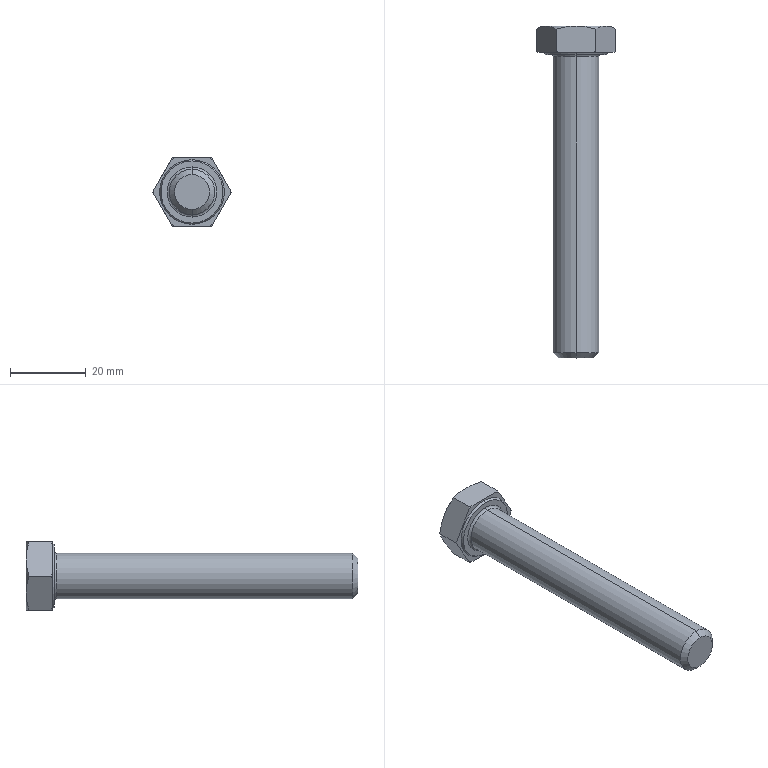Component | SolidWorks | GB_T5780-2016[HexHeadBoltGradeCM12_80]-1 | 1 solid | 30 faces | box 20.78 x 87.5 x 18 mm | volume 11078 mm3 | cone 16 | plane 10 | cylinder 2 | torus 2 | commonest cylinder face diameters 12 x2
build123d program:
from build123d import *

# Parameters (mm, degrees)
BASE_EXTRUDE_DEPTH = 7.5
CHAMFER_2_SIZE     = 1.4


with BuildPart() as part:
    # Sketch1 → Base-Extrude (new body)
    with BuildSketch(Plane(origin=(0, 0, 0), x_dir=(0, 0, -1), z_dir=(1, 0, 0))):
        Polygon((9, 5.196), (9, -5.196), (0, -10.392), (-9, -5.196), (-9, 5.196), (0, 10.392), align=None)
    extrude(amount=BASE_EXTRUDE_DEPTH)

    # Sketch2 → Revolve1 (revolve)
    with BuildSketch(Plane.XY, mode=Mode.PRIVATE) as revolve1_sk:
        Polygon((0, 0), (87.5, 0), (87.5, 4.484), (87.5, 6), (7.5, 6), (0, 6), align=None)
    revolve(revolve1_sk.sketch.rotate(Axis((0, 0, 0), (-1, 0, 0)), 90), axis=Axis((0, 0, 0), (-1, 0, 0)))

    # Sketch3 → Cut-Revolve1 (revolve, cut)
    with BuildSketch(Plane.XY):
        Polygon((0, 9), (3.691, 15.392), (3.691, 20.392), (-10, 20.392), (-10, 9), align=None)
    revolve(axis=Axis((0, 0, 0), (1, 0, 0)), mode=Mode.SUBTRACT)

    # Sketch5 → Cut-Revolve2 (revolve, cut)
    with BuildSketch(Plane.XY):
        Polygon((7.5, 9), (3.809, 15.392), (3.809, 20.392), (13.809, 20.392), (13.809, 9), align=None)
    revolve(axis=Axis((0, 0, 0), (1, 0, 0)), mode=Mode.SUBTRACT)

    # Sketch4 → Cut-Revolve3 (revolve, cut)
    with BuildSketch(Plane.XY, mode=Mode.PRIVATE) as cut_revolve3_sk:
        Polygon((7.5, 8.177), (6.9, 8.524), (6.9, 20.392), (7.5, 20.392), align=None)
    revolve(cut_revolve3_sk.sketch.rotate(Axis((0, 0, 0), (1, 0, 0)), 90), axis=Axis((0, 0, 0), (1, 0, 0)), mode=Mode.SUBTRACT)

    # Chamfer 2
    chamfer_2_edges = [part.edges().sort_by_distance(p)[0] for p in [
        (87.5, 0, 6),
    ]]
    chamfer(chamfer_2_edges, length=CHAMFER_2_SIZE)

    # Sketch9 → Revolve1_2 (revolve)
    with BuildSketch(Plane.XY, mode=Mode.PRIVATE) as revolve1_2_sk:
        with BuildLine():
            Line((7.5, 6.6), (7.5, 6))
            Line((7.5, 6), (8.1, 6))
            ThreePointArc((8.1, 6), (7.676, 6.176), (7.5, 6.6))
        make_face()
    revolve(revolve1_2_sk.sketch.rotate(Axis((0, 0, 0), (1, 0, 0)), 90), axis=Axis((0, 0, 0), (1, 0, 0)))


solid = part.part

# Placed as in the assembly
solid = solid.moved(Location((-380, 37.5, 90), (0, 0, -90)))
STEP:
#1=COLOUR_RGB('',0.7922,0.8196,0.9333);
#2=FILL_AREA_STYLE_COLOUR('',#1);
#3=FILL_AREA_STYLE('',(#2));
#4=SURFACE_STYLE_FILL_AREA(#3);
#5=SURFACE_SIDE_STYLE('',(#4));
#6=SURFACE_STYLE_USAGE(.BOTH.,#5);
#7=PRESENTATION_STYLE_ASSIGNMENT((#6));
#8=CARTESIAN_POINT('',(-14.961,1.157,3.78));
#9=VERTEX_POINT('',#8);
#10=CARTESIAN_POINT('',(-14.961,1.157,3.307));
#11=VERTEX_POINT('',#10);
#12=CARTESIAN_POINT('',(-14.961,1.157,3.543));
#13=DIRECTION('',(-0.,1.,0.));
#14=DIRECTION('',(0.,0.,1.));
#15=AXIS2_PLACEMENT_3D('',#12,#13,#14);
#16=CIRCLE('',#15,0.2362);
#17=EDGE_CURVE('',#9,#11,#16,.T.);
#18=ORIENTED_EDGE('',*,*,#17,.F.);
#19=CARTESIAN_POINT('',(-14.961,-1.913,3.78));
#20=VERTEX_POINT('',#19);
#21=CARTESIAN_POINT('',(-14.961,1.476,3.78));
#22=DIRECTION('',(0.,-1.,0.));
#23=VECTOR('',#22,39.37);
#24=LINE('',#21,#23);
#25=EDGE_CURVE('',#9,#20,#24,.T.);
#26=ORIENTED_EDGE('',*,*,#25,.T.);
#27=CARTESIAN_POINT('',(-14.961,-1.913,3.307));
#28=VERTEX_POINT('',#27);
#29=CARTESIAN_POINT('',(-14.961,-1.913,3.543));
#30=DIRECTION('',(-0.,1.,0.));
#31=DIRECTION('',(-0.,0.,-1.));
#32=AXIS2_PLACEMENT_3D('',#29,#30,#31);
#33=CIRCLE('',#32,0.2362);
#34=EDGE_CURVE('',#20,#28,#33,.T.);
#35=ORIENTED_EDGE('',*,*,#34,.T.);
#36=CARTESIAN_POINT('',(-14.961,1.476,3.307));
#37=DIRECTION('',(0.,-1.,0.));
#38=VECTOR('',#37,39.37);
#39=LINE('',#36,#38);
#40=EDGE_CURVE('',#11,#28,#39,.T.);
#41=ORIENTED_EDGE('',*,*,#40,.F.);
#42=EDGE_LOOP('',(#18,#26,#35,#41));
#43=FACE_OUTER_BOUND('',#42,.T.);
#44=CARTESIAN_POINT('',(-14.961,1.476,3.543));
#45=DIRECTION('',(0.,-1.,0.));
#46=DIRECTION('',(0.,0.,-1.));
#47=AXIS2_PLACEMENT_3D('',#44,#45,#46);
#48=CYLINDRICAL_SURFACE('',#47,0.2362);
#49=ADVANCED_FACE('',(#43),#48,.T.);
#50=CARTESIAN_POINT('',(-14.961,-1.969,3.362));
#51=VERTEX_POINT('',#50);
#52=CARTESIAN_POINT('',(-14.961,-1.969,3.724));
#53=VERTEX_POINT('',#52);
#54=CARTESIAN_POINT('',(-14.961,-1.969,3.543));
#55=DIRECTION('',(0.,-1.,0.));
#56=DIRECTION('',(0.,0.,-1.));
#57=AXIS2_PLACEMENT_3D('',#54,#55,#56);
#58=CIRCLE('',#57,0.1811);
#59=EDGE_CURVE('',#51,#53,#58,.T.);
#60=ORIENTED_EDGE('',*,*,#59,.F.);
#61=CARTESIAN_POINT('',(-14.961,-1.969,3.362));
#62=DIRECTION('',(-0.,0.7071,-0.7071));
#63=VECTOR('',#62,39.37);
#64=LINE('',#61,#63);
#65=EDGE_CURVE('',#51,#28,#64,.T.);
#66=ORIENTED_EDGE('',*,*,#65,.T.);
#67=ORIENTED_EDGE('',*,*,#34,.F.);
#68=CARTESIAN_POINT('',(-14.961,-1.969,3.724));
#69=DIRECTION('',(-0.,0.7071,0.7071));
#70=VECTOR('',#69,39.37);
#71=LINE('',#68,#70);
#72=EDGE_CURVE('',#53,#20,#71,.T.);
#73=ORIENTED_EDGE('',*,*,#72,.F.);
#74=EDGE_LOOP('',(#60,#66,#67,#73));
#75=FACE_OUTER_BOUND('',#74,.T.);
#76=CARTESIAN_POINT('',(-14.961,-1.969,3.543));
#77=DIRECTION('',(-0.,1.,0.));
#78=DIRECTION('',(0.,0.,1.));
#79=AXIS2_PLACEMENT_3D('',#76,#77,#78);
#80=CONICAL_SURFACE('',#79,0.1811,0.7854);
#81=ADVANCED_FACE('',(#75),#80,.T.);
#82=CARTESIAN_POINT('',(-14.961,1.181,3.283));
#83=VERTEX_POINT('',#82);
#84=CARTESIAN_POINT('',(-14.961,1.181,3.803));
#85=VERTEX_POINT('',#84);
#86=CARTESIAN_POINT('',(-14.961,1.181,3.543));
#87=DIRECTION('',(-0.,1.,0.));
#88=DIRECTION('',(0.,0.,1.));
#89=AXIS2_PLACEMENT_3D('',#86,#87,#88);
#90=CIRCLE('',#89,0.2598);
#91=EDGE_CURVE('',#83,#85,#90,.T.);
#92=ORIENTED_EDGE('',*,*,#91,.F.);
#93=CARTESIAN_POINT('',(-14.961,1.157,3.283));
#94=DIRECTION('',(1.,0.,0.));
#95=DIRECTION('',(0.,1.,0.));
#96=AXIS2_PLACEMENT_3D('',#93,#94,#95);
#97=CIRCLE('',#96,0.02362);
#98=EDGE_CURVE('',#83,#11,#97,.T.);
#99=ORIENTED_EDGE('',*,*,#98,.T.);
#100=CARTESIAN_POINT('',(-14.961,1.157,3.543));
#101=DIRECTION('',(-0.,1.,0.));
#102=DIRECTION('',(0.,0.,1.));
#103=AXIS2_PLACEMENT_3D('',#100,#101,#102);
#104=CIRCLE('',#103,0.2362);
#105=EDGE_CURVE('',#11,#9,#104,.T.);
#106=ORIENTED_EDGE('',*,*,#105,.T.);
#107=CARTESIAN_POINT('',(-14.961,1.157,3.803));
#108=DIRECTION('',(-1.,-0.,0.));
#109=DIRECTION('',(0.,-1.,0.));
#110=AXIS2_PLACEMENT_3D('',#107,#108,#109);
#111=CIRCLE('',#110,0.02362);
#112=EDGE_CURVE('',#85,#9,#111,.T.);
#113=ORIENTED_EDGE('',*,*,#112,.F.);
#114=EDGE_LOOP('',(#92,#99,#106,#113));
#115=FACE_OUTER_BOUND('',#114,.T.);
#116=CARTESIAN_POINT('',(-14.961,1.157,3.543));
#117=DIRECTION('',(-0.,1.,0.));
#118=DIRECTION('',(0.,0.,1.));
#119=AXIS2_PLACEMENT_3D('',#116,#117,#118);
#120=TOROIDAL_SURFACE('',#119,0.2598,0.02362);
#121=ADVANCED_FACE('',(#115),#120,.F.);
#122=CARTESIAN_POINT('',(-14.961,1.181,3.865));
#123=VERTEX_POINT('',#122);
#124=CARTESIAN_POINT('',(-14.961,1.181,3.221));
#125=VERTEX_POINT('',#124);
#126=CARTESIAN_POINT('',(-14.961,1.181,3.543));
#127=DIRECTION('',(-0.,1.,0.));
#128=DIRECTION('',(0.,0.,1.));
#129=AXIS2_PLACEMENT_3D('',#126,#127,#128);
#130=CIRCLE('',#129,0.3219);
#131=EDGE_CURVE('',#123,#125,#130,.T.);
#132=ORIENTED_EDGE('',*,*,#131,.T.);
#133=CARTESIAN_POINT('',(-14.961,1.205,3.208));
#134=VERTEX_POINT('',#133);
#135=CARTESIAN_POINT('',(-14.961,1.205,3.208));
#136=DIRECTION('',(-0.,0.866,-0.5));
#137=VECTOR('',#136,39.37);
#138=LINE('',#135,#137);
#139=EDGE_CURVE('',#125,#134,#138,.T.);
#140=ORIENTED_EDGE('',*,*,#139,.T.);
#141=CARTESIAN_POINT('',(-14.961,1.205,3.879));
#142=VERTEX_POINT('',#141);
#143=CARTESIAN_POINT('',(-14.961,1.205,3.543));
#144=DIRECTION('',(-0.,1.,0.));
#145=DIRECTION('',(0.,0.,1.));
#146=AXIS2_PLACEMENT_3D('',#143,#144,#145);
#147=CIRCLE('',#146,0.3356);
#148=EDGE_CURVE('',#142,#134,#147,.T.);
#149=ORIENTED_EDGE('',*,*,#148,.F.);
#150=CARTESIAN_POINT('',(-14.961,1.205,3.879));
#151=DIRECTION('',(-0.,0.866,0.5));
#152=VECTOR('',#151,39.37);
#153=LINE('',#150,#152);
#154=EDGE_CURVE('',#123,#142,#153,.T.);
#155=ORIENTED_EDGE('',*,*,#154,.F.);
#156=EDGE_LOOP('',(#132,#140,#149,#155));
#157=FACE_OUTER_BOUND('',#156,.T.);
#158=CARTESIAN_POINT('',(-14.961,1.205,3.543));
#159=DIRECTION('',(-0.,1.,0.));
#160=DIRECTION('',(0.,0.,1.));
#161=AXIS2_PLACEMENT_3D('',#158,#159,#160);
#162=CONICAL_SURFACE('',#161,0.3356,0.5236);
#163=ADVANCED_FACE('',(#157),#162,.T.);
#164=ORIENTED_EDGE('',*,*,#131,.F.);
#165=CARTESIAN_POINT('',(-14.961,1.181,3.543));
#166=DIRECTION('',(-0.,1.,0.));
#167=DIRECTION('',(0.,0.,1.));
#168=AXIS2_PLACEMENT_3D('',#165,#166,#167);
#169=CIRCLE('',#168,0.3219);
#170=EDGE_CURVE('',#125,#123,#169,.T.);
#171=ORIENTED_EDGE('',*,*,#170,.F.);
#172=EDGE_LOOP('',(#164,#171));
#173=FACE_OUTER_BOUND('',#172,.T.);
#174=CARTESIAN_POINT('',(-14.961,1.181,3.543));
#175=DIRECTION('',(-0.,1.,0.));
#176=DIRECTION('',(0.,0.,1.));
#177=AXIS2_PLACEMENT_3D('',#174,#175,#176);
#178=CIRCLE('',#177,0.2598);
#179=EDGE_CURVE('',#85,#83,#178,.T.);
#180=ORIENTED_EDGE('',*,*,#179,.T.);
#181=ORIENTED_EDGE('',*,*,#91,.T.);
#182=EDGE_LOOP('',(#180,#181));
#183=FACE_BOUND('',#182,.T.);
#184=CARTESIAN_POINT('',(-14.551,1.181,3.543));
#185=DIRECTION('',(0.,-1.,0.));
#186=DIRECTION('',(0.,0.,-1.));
#187=AXIS2_PLACEMENT_3D('',#184,#185,#186);
#188=PLANE('',#187);
#189=ADVANCED_FACE('',(#173,#183),#188,.T.);
#190=CARTESIAN_POINT('',(-14.741,1.205,3.214));
#191=VERTEX_POINT('',#190);
#192=CARTESIAN_POINT('',(-14.566,1.205,3.518));
#193=VERTEX_POINT('',#192);
#194=CARTESIAN_POINT('',(-14.756,1.205,3.189));
#195=DIRECTION('',(0.5,0.,0.866));
#196=VECTOR('',#195,39.37);
#197=LINE('',#194,#196);
#198=EDGE_CURVE('',#191,#193,#197,.T.);
#199=ORIENTED_EDGE('',*,*,#198,.F.);
#200=CARTESIAN_POINT('',(-14.756,1.213,3.189));
#201=VERTEX_POINT('',#200);
#202=CARTESIAN_POINT('',(-14.756,1.213,3.189));
#203=CARTESIAN_POINT('',(-14.751,1.21,3.197));
#204=CARTESIAN_POINT('',(-14.746,1.207,3.206));
#205=CARTESIAN_POINT('',(-14.741,1.205,3.214));
#206=B_SPLINE_CURVE_WITH_KNOTS('',3,(#202,#203,#204,#205),.UNSPECIFIED.,.F.,.F.,(4,4),(0.00000024,0.0007696),.UNSPECIFIED.);
#207=EDGE_CURVE('',#201,#191,#206,.T.);
#208=ORIENTED_EDGE('',*,*,#207,.F.);
#209=CARTESIAN_POINT('',(-14.756,1.445,3.189));
#210=VERTEX_POINT('',#209);
#211=CARTESIAN_POINT('',(-14.756,1.181,3.189));
#212=DIRECTION('',(-0.,1.,0.));
#213=VECTOR('',#212,39.37);
#214=LINE('',#211,#213);
#215=EDGE_CURVE('',#201,#210,#214,.T.);
#216=ORIENTED_EDGE('',*,*,#215,.T.);
#217=CARTESIAN_POINT('',(-14.654,1.476,3.366));
#218=VERTEX_POINT('',#217);
#219=CARTESIAN_POINT('',(-14.654,1.476,3.366));
#220=CARTESIAN_POINT('',(-14.662,1.476,3.351));
#221=CARTESIAN_POINT('',(-14.671,1.476,3.336));
#222=CARTESIAN_POINT('',(-14.688,1.473,3.306));
#223=CARTESIAN_POINT('',(-14.697,1.471,3.291));
#224=CARTESIAN_POINT('',(-14.723,1.462,3.247));
#225=CARTESIAN_POINT('',(-14.739,1.454,3.218));
#226=CARTESIAN_POINT('',(-14.756,1.445,3.189));
#227=B_SPLINE_CURVE_WITH_KNOTS('',3,(#219,#220,#221,#222,#223,#224,#225,#226),.UNSPECIFIED.,.F.,.F.,(4,2,2,4),(0.005258,0.006567,0.007877,0.0105),.UNSPECIFIED.);
#228=EDGE_CURVE('',#218,#210,#227,.T.);
#229=ORIENTED_EDGE('',*,*,#228,.F.);
#230=CARTESIAN_POINT('',(-14.551,1.445,3.543));
#231=VERTEX_POINT('',#230);
#232=CARTESIAN_POINT('',(-14.551,1.445,3.543));
#233=CARTESIAN_POINT('',(-14.568,1.454,3.514));
#234=CARTESIAN_POINT('',(-14.585,1.462,3.485));
#235=CARTESIAN_POINT('',(-14.619,1.473,3.426));
#236=CARTESIAN_POINT('',(-14.636,1.476,3.396));
#237=CARTESIAN_POINT('',(-14.654,1.476,3.366));
#238=B_SPLINE_CURVE_WITH_KNOTS('',3,(#232,#233,#234,#235,#236,#237),.UNSPECIFIED.,.F.,.F.,(4,2,4),(0.00000024,0.002629,0.005258),.UNSPECIFIED.);
#239=EDGE_CURVE('',#231,#218,#238,.T.);
#240=ORIENTED_EDGE('',*,*,#239,.F.);
#241=CARTESIAN_POINT('',(-14.551,1.213,3.543));
#242=VERTEX_POINT('',#241);
#243=CARTESIAN_POINT('',(-14.551,1.181,3.543));
#244=DIRECTION('',(-0.,1.,0.));
#245=VECTOR('',#244,39.37);
#246=LINE('',#243,#245);
#247=EDGE_CURVE('',#242,#231,#246,.T.);
#248=ORIENTED_EDGE('',*,*,#247,.F.);
#249=CARTESIAN_POINT('',(-14.566,1.205,3.518));
#250=CARTESIAN_POINT('',(-14.561,1.207,3.526));
#251=CARTESIAN_POINT('',(-14.556,1.21,3.535));
#252=CARTESIAN_POINT('',(-14.551,1.213,3.543));
#253=B_SPLINE_CURVE_WITH_KNOTS('',3,(#249,#250,#251,#252),.UNSPECIFIED.,.F.,.F.,(4,4),(0.009728,0.0105),.UNSPECIFIED.);
#254=EDGE_CURVE('',#193,#242,#253,.T.);
#255=ORIENTED_EDGE('',*,*,#254,.F.);
#256=EDGE_LOOP('',(#199,#208,#216,#229,#240,#248,#255));
#257=FACE_OUTER_BOUND('',#256,.T.);
#258=CARTESIAN_POINT('',(-14.756,1.181,3.189));
#259=DIRECTION('',(-0.866,-0.,0.5));
#260=DIRECTION('',(-0.5,-0.,-0.866));
#261=AXIS2_PLACEMENT_3D('',#258,#259,#260);
#262=PLANE('',#261);
#263=ADVANCED_FACE('',(#257),#262,.F.);
#264=CARTESIAN_POINT('',(-14.566,1.205,3.569));
#265=VERTEX_POINT('',#264);
#266=CARTESIAN_POINT('',(-14.741,1.205,3.872));
#267=VERTEX_POINT('',#266);
#268=CARTESIAN_POINT('',(-14.551,1.205,3.543));
#269=DIRECTION('',(-0.5,-0.,0.866));
#270=VECTOR('',#269,39.37);
#271=LINE('',#268,#270);
#272=EDGE_CURVE('',#265,#267,#271,.T.);
#273=ORIENTED_EDGE('',*,*,#272,.F.);
#274=CARTESIAN_POINT('',(-14.551,1.213,3.543));
#275=CARTESIAN_POINT('',(-14.556,1.21,3.552));
#276=CARTESIAN_POINT('',(-14.561,1.207,3.56));
#277=CARTESIAN_POINT('',(-14.566,1.205,3.569));
#278=B_SPLINE_CURVE_WITH_KNOTS('',3,(#274,#275,#276,#277),.UNSPECIFIED.,.F.,.F.,(4,4),(0.00000024,0.0007696),.UNSPECIFIED.);
#279=EDGE_CURVE('',#242,#265,#278,.T.);
#280=ORIENTED_EDGE('',*,*,#279,.F.);
#281=ORIENTED_EDGE('',*,*,#247,.T.);
#282=CARTESIAN_POINT('',(-14.654,1.476,3.72));
#283=VERTEX_POINT('',#282);
#284=CARTESIAN_POINT('',(-14.654,1.476,3.72));
#285=CARTESIAN_POINT('',(-14.645,1.476,3.705));
#286=CARTESIAN_POINT('',(-14.636,1.476,3.69));
#287=CARTESIAN_POINT('',(-14.619,1.473,3.66));
#288=CARTESIAN_POINT('',(-14.611,1.471,3.646));
#289=CARTESIAN_POINT('',(-14.585,1.462,3.601));
#290=CARTESIAN_POINT('',(-14.568,1.454,3.572));
#291=CARTESIAN_POINT('',(-14.551,1.445,3.543));
#292=B_SPLINE_CURVE_WITH_KNOTS('',3,(#284,#285,#286,#287,#288,#289,#290,#291),.UNSPECIFIED.,.F.,.F.,(4,2,2,4),(0.005258,0.006567,0.007877,0.0105),.UNSPECIFIED.);
#293=EDGE_CURVE('',#283,#231,#292,.T.);
#294=ORIENTED_EDGE('',*,*,#293,.F.);
#295=CARTESIAN_POINT('',(-14.756,1.445,3.898));
#296=VERTEX_POINT('',#295);
#297=CARTESIAN_POINT('',(-14.756,1.445,3.898));
#298=CARTESIAN_POINT('',(-14.739,1.454,3.869));
#299=CARTESIAN_POINT('',(-14.722,1.462,3.839));
#300=CARTESIAN_POINT('',(-14.688,1.473,3.78));
#301=CARTESIAN_POINT('',(-14.671,1.476,3.751));
#302=CARTESIAN_POINT('',(-14.654,1.476,3.72));
#303=B_SPLINE_CURVE_WITH_KNOTS('',3,(#297,#298,#299,#300,#301,#302),.UNSPECIFIED.,.F.,.F.,(4,2,4),(0.00000024,0.002629,0.005258),.UNSPECIFIED.);
#304=EDGE_CURVE('',#296,#283,#303,.T.);
#305=ORIENTED_EDGE('',*,*,#304,.F.);
#306=CARTESIAN_POINT('',(-14.756,1.213,3.898));
#307=VERTEX_POINT('',#306);
#308=CARTESIAN_POINT('',(-14.756,1.181,3.898));
#309=DIRECTION('',(-0.,1.,0.));
#310=VECTOR('',#309,39.37);
#311=LINE('',#308,#310);
#312=EDGE_CURVE('',#307,#296,#311,.T.);
#313=ORIENTED_EDGE('',*,*,#312,.F.);
#314=CARTESIAN_POINT('',(-14.741,1.205,3.872));
#315=CARTESIAN_POINT('',(-14.746,1.207,3.881));
#316=CARTESIAN_POINT('',(-14.751,1.21,3.889));
#317=CARTESIAN_POINT('',(-14.756,1.213,3.898));
#318=B_SPLINE_CURVE_WITH_KNOTS('',3,(#314,#315,#316,#317),.UNSPECIFIED.,.F.,.F.,(4,4),(0.009728,0.0105),.UNSPECIFIED.);
#319=EDGE_CURVE('',#267,#307,#318,.T.);
#320=ORIENTED_EDGE('',*,*,#319,.F.);
#321=EDGE_LOOP('',(#273,#280,#281,#294,#305,#313,#320));
#322=FACE_OUTER_BOUND('',#321,.T.);
#323=CARTESIAN_POINT('',(-14.551,1.181,3.543));
#324=DIRECTION('',(-0.866,-0.,-0.5));
#325=DIRECTION('',(0.5,0.,-0.866));
#326=AXIS2_PLACEMENT_3D('',#323,#324,#325);
#327=PLANE('',#326);
#328=ADVANCED_FACE('',(#322),#327,.F.);
#329=CARTESIAN_POINT('',(-14.786,1.205,3.898));
#330=VERTEX_POINT('',#329);
#331=CARTESIAN_POINT('',(-15.136,1.205,3.898));
#332=VERTEX_POINT('',#331);
#333=CARTESIAN_POINT('',(-14.756,1.205,3.898));
#334=DIRECTION('',(-1.,-0.,-0.));
#335=VECTOR('',#334,39.37);
#336=LINE('',#333,#335);
#337=EDGE_CURVE('',#330,#332,#336,.T.);
#338=ORIENTED_EDGE('',*,*,#337,.F.);
#339=CARTESIAN_POINT('',(-14.756,1.213,3.898));
#340=CARTESIAN_POINT('',(-14.766,1.21,3.898));
#341=CARTESIAN_POINT('',(-14.776,1.207,3.898));
#342=CARTESIAN_POINT('',(-14.786,1.205,3.898));
#343=B_SPLINE_CURVE_WITH_KNOTS('',3,(#339,#340,#341,#342),.UNSPECIFIED.,.F.,.F.,(4,4),(0.02519,0.02597),.UNSPECIFIED.);
#344=EDGE_CURVE('',#307,#330,#343,.T.);
#345=ORIENTED_EDGE('',*,*,#344,.F.);
#346=ORIENTED_EDGE('',*,*,#312,.T.);
#347=CARTESIAN_POINT('',(-14.961,1.476,3.898));
#348=VERTEX_POINT('',#347);
#349=CARTESIAN_POINT('',(-14.961,1.476,3.898));
#350=CARTESIAN_POINT('',(-14.943,1.476,3.898));
#351=CARTESIAN_POINT('',(-14.926,1.476,3.898));
#352=CARTESIAN_POINT('',(-14.891,1.473,3.898));
#353=CARTESIAN_POINT('',(-14.874,1.471,3.898));
#354=CARTESIAN_POINT('',(-14.823,1.462,3.898));
#355=CARTESIAN_POINT('',(-14.789,1.454,3.898));
#356=CARTESIAN_POINT('',(-14.756,1.445,3.898));
#357=B_SPLINE_CURVE_WITH_KNOTS('',3,(#349,#350,#351,#352,#353,#354,#355,#356),.UNSPECIFIED.,.F.,.F.,(4,2,2,4),(0.01498,0.0163,0.01761,0.02025),.UNSPECIFIED.);
#358=EDGE_CURVE('',#348,#296,#357,.T.);
#359=ORIENTED_EDGE('',*,*,#358,.F.);
#360=CARTESIAN_POINT('',(-15.165,1.445,3.898));
#361=VERTEX_POINT('',#360);
#362=CARTESIAN_POINT('',(-15.165,1.445,3.898));
#363=CARTESIAN_POINT('',(-15.132,1.454,3.898));
#364=CARTESIAN_POINT('',(-15.098,1.462,3.898));
#365=CARTESIAN_POINT('',(-15.03,1.473,3.898));
#366=CARTESIAN_POINT('',(-14.995,1.476,3.898));
#367=CARTESIAN_POINT('',(-14.961,1.476,3.898));
#368=B_SPLINE_CURVE_WITH_KNOTS('',3,(#362,#363,#364,#365,#366,#367),.UNSPECIFIED.,.F.,.F.,(4,2,4),(0.00972,0.01235,0.01498),.UNSPECIFIED.);
#369=EDGE_CURVE('',#361,#348,#368,.T.);
#370=ORIENTED_EDGE('',*,*,#369,.F.);
#371=CARTESIAN_POINT('',(-15.165,1.213,3.898));
#372=VERTEX_POINT('',#371);
#373=CARTESIAN_POINT('',(-15.165,1.181,3.898));
#374=DIRECTION('',(-0.,1.,0.));
#375=VECTOR('',#374,39.37);
#376=LINE('',#373,#375);
#377=EDGE_CURVE('',#372,#361,#376,.T.);
#378=ORIENTED_EDGE('',*,*,#377,.F.);
#379=CARTESIAN_POINT('',(-15.136,1.205,3.898));
#380=CARTESIAN_POINT('',(-15.146,1.207,3.898));
#381=CARTESIAN_POINT('',(-15.155,1.21,3.898));
#382=CARTESIAN_POINT('',(-15.165,1.213,3.898));
#383=B_SPLINE_CURVE_WITH_KNOTS('',3,(#379,#380,#381,#382),.UNSPECIFIED.,.F.,.F.,(4,4),(0.03494,0.03571),.UNSPECIFIED.);
#384=EDGE_CURVE('',#332,#372,#383,.T.);
#385=ORIENTED_EDGE('',*,*,#384,.F.);
#386=EDGE_LOOP('',(#338,#345,#346,#359,#370,#378,#385));
#387=FACE_OUTER_BOUND('',#386,.T.);
#388=CARTESIAN_POINT('',(-14.756,1.181,3.898));
#389=DIRECTION('',(0.,0.,-1.));
#390=DIRECTION('',(1.,0.,0.));
#391=AXIS2_PLACEMENT_3D('',#388,#389,#390);
#392=PLANE('',#391);
#393=ADVANCED_FACE('',(#387),#392,.F.);
#394=CARTESIAN_POINT('',(-15.18,1.205,3.872));
#395=VERTEX_POINT('',#394);
#396=CARTESIAN_POINT('',(-15.355,1.205,3.569));
#397=VERTEX_POINT('',#396);
#398=CARTESIAN_POINT('',(-15.37,1.205,3.543));
#399=DIRECTION('',(-0.5,-0.,-0.866));
#400=VECTOR('',#399,39.37);
#401=LINE('',#398,#400);
#402=EDGE_CURVE('',#395,#397,#401,.T.);
#403=ORIENTED_EDGE('',*,*,#402,.F.);
#404=CARTESIAN_POINT('',(-15.165,1.213,3.898));
#405=CARTESIAN_POINT('',(-15.17,1.21,3.889));
#406=CARTESIAN_POINT('',(-15.175,1.207,3.881));
#407=CARTESIAN_POINT('',(-15.18,1.205,3.872));
#408=B_SPLINE_CURVE_WITH_KNOTS('',3,(#404,#405,#406,#407),.UNSPECIFIED.,.F.,.F.,(4,4),(0.00000024,0.0007696),.UNSPECIFIED.);
#409=EDGE_CURVE('',#372,#395,#408,.T.);
#410=ORIENTED_EDGE('',*,*,#409,.F.);
#411=ORIENTED_EDGE('',*,*,#377,.T.);
#412=CARTESIAN_POINT('',(-15.267,1.476,3.72));
#413=VERTEX_POINT('',#412);
#414=CARTESIAN_POINT('',(-15.267,1.476,3.72));
#415=CARTESIAN_POINT('',(-15.259,1.476,3.736));
#416=CARTESIAN_POINT('',(-15.25,1.476,3.751));
#417=CARTESIAN_POINT('',(-15.233,1.473,3.78));
#418=CARTESIAN_POINT('',(-15.224,1.471,3.795));
#419=CARTESIAN_POINT('',(-15.199,1.462,3.84));
#420=CARTESIAN_POINT('',(-15.182,1.454,3.869));
#421=CARTESIAN_POINT('',(-15.165,1.445,3.898));
#422=B_SPLINE_CURVE_WITH_KNOTS('',3,(#414,#415,#416,#417,#418,#419,#420,#421),.UNSPECIFIED.,.F.,.F.,(4,2,2,4),(0.005258,0.006567,0.007877,0.0105),.UNSPECIFIED.);
#423=EDGE_CURVE('',#413,#361,#422,.T.);
#424=ORIENTED_EDGE('',*,*,#423,.F.);
#425=CARTESIAN_POINT('',(-15.37,1.445,3.543));
#426=VERTEX_POINT('',#425);
#427=CARTESIAN_POINT('',(-15.37,1.445,3.543));
#428=CARTESIAN_POINT('',(-15.353,1.454,3.572));
#429=CARTESIAN_POINT('',(-15.336,1.462,3.601));
#430=CARTESIAN_POINT('',(-15.302,1.473,3.66));
#431=CARTESIAN_POINT('',(-15.285,1.476,3.69));
#432=CARTESIAN_POINT('',(-15.267,1.476,3.72));
#433=B_SPLINE_CURVE_WITH_KNOTS('',3,(#427,#428,#429,#430,#431,#432),.UNSPECIFIED.,.F.,.F.,(4,2,4),(0.00000024,0.002629,0.005258),.UNSPECIFIED.);
#434=EDGE_CURVE('',#426,#413,#433,.T.);
#435=ORIENTED_EDGE('',*,*,#434,.F.);
#436=CARTESIAN_POINT('',(-15.37,1.213,3.543));
#437=VERTEX_POINT('',#436);
#438=CARTESIAN_POINT('',(-15.37,1.181,3.543));
#439=DIRECTION('',(-0.,1.,0.));
#440=VECTOR('',#439,39.37);
#441=LINE('',#438,#440);
#442=EDGE_CURVE('',#437,#426,#441,.T.);
#443=ORIENTED_EDGE('',*,*,#442,.F.);
#444=CARTESIAN_POINT('',(-15.355,1.205,3.569));
#445=CARTESIAN_POINT('',(-15.36,1.207,3.56));
#446=CARTESIAN_POINT('',(-15.365,1.21,3.552));
#447=CARTESIAN_POINT('',(-15.37,1.213,3.543));
#448=B_SPLINE_CURVE_WITH_KNOTS('',3,(#444,#445,#446,#447),.UNSPECIFIED.,.F.,.F.,(4,4),(0.009728,0.0105),.UNSPECIFIED.);
#449=EDGE_CURVE('',#397,#437,#448,.T.);
#450=ORIENTED_EDGE('',*,*,#449,.F.);
#451=EDGE_LOOP('',(#403,#410,#411,#424,#435,#443,#450));
#452=FACE_OUTER_BOUND('',#451,.T.);
#453=CARTESIAN_POINT('',(-15.37,1.181,3.543));
#454=DIRECTION('',(0.866,0.,-0.5));
#455=DIRECTION('',(0.5,0.,0.866));
#456=AXIS2_PLACEMENT_3D('',#453,#454,#455);
#457=PLANE('',#456);
#458=ADVANCED_FACE('',(#452),#457,.F.);
#459=CARTESIAN_POINT('',(-15.355,1.205,3.518));
#460=VERTEX_POINT('',#459);
#461=CARTESIAN_POINT('',(-15.18,1.205,3.214));
#462=VERTEX_POINT('',#461);
#463=CARTESIAN_POINT('',(-15.165,1.205,3.189));
#464=DIRECTION('',(0.5,0.,-0.866));
#465=VECTOR('',#464,39.37);
#466=LINE('',#463,#465);
#467=EDGE_CURVE('',#460,#462,#466,.T.);
#468=ORIENTED_EDGE('',*,*,#467,.F.);
#469=CARTESIAN_POINT('',(-15.37,1.213,3.543));
#470=CARTESIAN_POINT('',(-15.365,1.21,3.535));
#471=CARTESIAN_POINT('',(-15.36,1.207,3.526));
#472=CARTESIAN_POINT('',(-15.355,1.205,3.518));
#473=B_SPLINE_CURVE_WITH_KNOTS('',3,(#469,#470,#471,#472),.UNSPECIFIED.,.F.,.F.,(4,4),(0.00000024,0.0007696),.UNSPECIFIED.);
#474=EDGE_CURVE('',#437,#460,#473,.T.);
#475=ORIENTED_EDGE('',*,*,#474,.F.);
#476=ORIENTED_EDGE('',*,*,#442,.T.);
#477=CARTESIAN_POINT('',(-15.267,1.476,3.366));
#478=VERTEX_POINT('',#477);
#479=CARTESIAN_POINT('',(-15.267,1.476,3.366));
#480=CARTESIAN_POINT('',(-15.276,1.476,3.381));
#481=CARTESIAN_POINT('',(-15.285,1.476,3.396));
#482=CARTESIAN_POINT('',(-15.302,1.473,3.426));
#483=CARTESIAN_POINT('',(-15.311,1.471,3.441));
#484=CARTESIAN_POINT('',(-15.336,1.462,3.485));
#485=CARTESIAN_POINT('',(-15.353,1.454,3.514));
#486=CARTESIAN_POINT('',(-15.37,1.445,3.543));
#487=B_SPLINE_CURVE_WITH_KNOTS('',3,(#479,#480,#481,#482,#483,#484,#485,#486),.UNSPECIFIED.,.F.,.F.,(4,2,2,4),(0.005258,0.006567,0.007877,0.0105),.UNSPECIFIED.);
#488=EDGE_CURVE('',#478,#426,#487,.T.);
#489=ORIENTED_EDGE('',*,*,#488,.F.);
#490=CARTESIAN_POINT('',(-15.165,1.445,3.189));
#491=VERTEX_POINT('',#490);
#492=CARTESIAN_POINT('',(-15.165,1.445,3.189));
#493=CARTESIAN_POINT('',(-15.182,1.454,3.218));
#494=CARTESIAN_POINT('',(-15.199,1.462,3.247));
#495=CARTESIAN_POINT('',(-15.233,1.473,3.306));
#496=CARTESIAN_POINT('',(-15.25,1.476,3.336));
#497=CARTESIAN_POINT('',(-15.267,1.476,3.366));
#498=B_SPLINE_CURVE_WITH_KNOTS('',3,(#492,#493,#494,#495,#496,#497),.UNSPECIFIED.,.F.,.F.,(4,2,4),(0.00000024,0.002629,0.005258),.UNSPECIFIED.);
#499=EDGE_CURVE('',#491,#478,#498,.T.);
#500=ORIENTED_EDGE('',*,*,#499,.F.);
#501=CARTESIAN_POINT('',(-15.165,1.213,3.189));
#502=VERTEX_POINT('',#501);
#503=CARTESIAN_POINT('',(-15.165,1.181,3.189));
#504=DIRECTION('',(-0.,1.,0.));
#505=VECTOR('',#504,39.37);
#506=LINE('',#503,#505);
#507=EDGE_CURVE('',#502,#491,#506,.T.);
#508=ORIENTED_EDGE('',*,*,#507,.F.);
#509=CARTESIAN_POINT('',(-15.18,1.205,3.214));
#510=CARTESIAN_POINT('',(-15.175,1.207,3.206));
#511=CARTESIAN_POINT('',(-15.17,1.21,3.197));
#512=CARTESIAN_POINT('',(-15.165,1.213,3.189));
#513=B_SPLINE_CURVE_WITH_KNOTS('',3,(#509,#510,#511,#512),.UNSPECIFIED.,.F.,.F.,(4,4),(0.009728,0.0105),.UNSPECIFIED.);
#514=EDGE_CURVE('',#462,#502,#513,.T.);
#515=ORIENTED_EDGE('',*,*,#514,.F.);
#516=EDGE_LOOP('',(#468,#475,#476,#489,#500,#508,#515));
#517=FACE_OUTER_BOUND('',#516,.T.);
#518=CARTESIAN_POINT('',(-15.165,1.181,3.189));
#519=DIRECTION('',(0.866,0.,0.5));
#520=DIRECTION('',(-0.5,-0.,0.866));
#521=AXIS2_PLACEMENT_3D('',#518,#519,#520);
#522=PLANE('',#521);
#523=ADVANCED_FACE('',(#517),#522,.F.);
#524=CARTESIAN_POINT('',(-15.136,1.205,3.189));
#525=VERTEX_POINT('',#524);
#526=CARTESIAN_POINT('',(-14.786,1.205,3.189));
#527=VERTEX_POINT('',#526);
#528=CARTESIAN_POINT('',(-14.756,1.205,3.189));
#529=DIRECTION('',(1.,0.,0.));
#530=VECTOR('',#529,39.37);
#531=LINE('',#528,#530);
#532=EDGE_CURVE('',#525,#527,#531,.T.);
#533=ORIENTED_EDGE('',*,*,#532,.F.);
#534=CARTESIAN_POINT('',(-15.165,1.213,3.189));
#535=CARTESIAN_POINT('',(-15.155,1.21,3.189));
#536=CARTESIAN_POINT('',(-15.146,1.207,3.189));
#537=CARTESIAN_POINT('',(-15.136,1.205,3.189));
#538=B_SPLINE_CURVE_WITH_KNOTS('',3,(#534,#535,#536,#537),.UNSPECIFIED.,.F.,.F.,(4,4),(0.00972,0.01049),.UNSPECIFIED.);
#539=EDGE_CURVE('',#502,#525,#538,.T.);
#540=ORIENTED_EDGE('',*,*,#539,.F.);
#541=ORIENTED_EDGE('',*,*,#507,.T.);
#542=CARTESIAN_POINT('',(-14.961,1.476,3.189));
#543=VERTEX_POINT('',#542);
#544=CARTESIAN_POINT('',(-14.961,1.476,3.189));
#545=CARTESIAN_POINT('',(-14.995,1.476,3.189));
#546=CARTESIAN_POINT('',(-15.03,1.473,3.189));
#547=CARTESIAN_POINT('',(-15.098,1.462,3.189));
#548=CARTESIAN_POINT('',(-15.132,1.454,3.189));
#549=CARTESIAN_POINT('',(-15.165,1.445,3.189));
#550=B_SPLINE_CURVE_WITH_KNOTS('',3,(#544,#545,#546,#547,#548,#549),.UNSPECIFIED.,.F.,.F.,(4,2,4),(0.03045,0.03308,0.03571),.UNSPECIFIED.);
#551=EDGE_CURVE('',#543,#491,#550,.T.);
#552=ORIENTED_EDGE('',*,*,#551,.F.);
#553=CARTESIAN_POINT('',(-14.756,1.445,3.189));
#554=CARTESIAN_POINT('',(-14.789,1.454,3.189));
#555=CARTESIAN_POINT('',(-14.823,1.462,3.189));
#556=CARTESIAN_POINT('',(-14.874,1.471,3.189));
#557=CARTESIAN_POINT('',(-14.891,1.473,3.189));
#558=CARTESIAN_POINT('',(-14.926,1.476,3.189));
#559=CARTESIAN_POINT('',(-14.943,1.476,3.189));
#560=CARTESIAN_POINT('',(-14.961,1.476,3.189));
#561=B_SPLINE_CURVE_WITH_KNOTS('',3,(#553,#554,#555,#556,#557,#558,#559,#560),.UNSPECIFIED.,.F.,.F.,(4,2,2,4),(0.02519,0.02782,0.02914,0.03045),.UNSPECIFIED.);
#562=EDGE_CURVE('',#210,#543,#561,.T.);
#563=ORIENTED_EDGE('',*,*,#562,.F.);
#564=ORIENTED_EDGE('',*,*,#215,.F.);
#565=CARTESIAN_POINT('',(-14.786,1.205,3.189));
#566=CARTESIAN_POINT('',(-14.776,1.207,3.189));
#567=CARTESIAN_POINT('',(-14.766,1.21,3.189));
#568=CARTESIAN_POINT('',(-14.756,1.213,3.189));
#569=B_SPLINE_CURVE_WITH_KNOTS('',3,(#565,#566,#567,#568),.UNSPECIFIED.,.F.,.F.,(4,4),(0.01947,0.02025),.UNSPECIFIED.);
#570=EDGE_CURVE('',#527,#201,#569,.T.);
#571=ORIENTED_EDGE('',*,*,#570,.F.);
#572=EDGE_LOOP('',(#533,#540,#541,#552,#563,#564,#571));
#573=FACE_OUTER_BOUND('',#572,.T.);
#574=CARTESIAN_POINT('',(-14.756,1.181,3.189));
#575=DIRECTION('',(0.,0.,1.));
#576=DIRECTION('',(0.,-1.,0.));
#577=AXIS2_PLACEMENT_3D('',#574,#575,#576);
#578=PLANE('',#577);
#579=ADVANCED_FACE('',(#573),#578,.F.);
#580=ORIENTED_EDGE('',*,*,#539,.T.);
#581=CARTESIAN_POINT('',(-14.961,1.205,3.543));
#582=DIRECTION('',(-0.,1.,0.));
#583=DIRECTION('',(0.,0.,-1.));
#584=AXIS2_PLACEMENT_3D('',#581,#582,#583);
#585=CIRCLE('',#584,0.3952);
#586=EDGE_CURVE('',#525,#462,#585,.T.);
#587=ORIENTED_EDGE('',*,*,#586,.T.);
#588=ORIENTED_EDGE('',*,*,#514,.T.);
#589=EDGE_LOOP('',(#580,#587,#588));
#590=FACE_OUTER_BOUND('',#589,.T.);
#591=CARTESIAN_POINT('',(-14.961,1.326,3.543));
#592=DIRECTION('',(-0.,1.,0.));
#593=DIRECTION('',(0.,0.,1.));
#594=AXIS2_PLACEMENT_3D('',#591,#592,#593);
#595=CONICAL_SURFACE('',#594,0.606,1.047);
#596=ADVANCED_FACE('',(#590),#595,.T.);
#597=ORIENTED_EDGE('',*,*,#474,.T.);
#598=CARTESIAN_POINT('',(-14.961,1.205,3.543));
#599=DIRECTION('',(-0.,1.,0.));
#600=DIRECTION('',(-0.,0.,-1.));
#601=AXIS2_PLACEMENT_3D('',#598,#599,#600);
#602=CIRCLE('',#601,0.3952);
#603=EDGE_CURVE('',#460,#397,#602,.T.);
#604=ORIENTED_EDGE('',*,*,#603,.T.);
#605=ORIENTED_EDGE('',*,*,#449,.T.);
#606=EDGE_LOOP('',(#597,#604,#605));
#607=FACE_OUTER_BOUND('',#606,.T.);
#608=CARTESIAN_POINT('',(-14.961,1.326,3.543));
#609=DIRECTION('',(-0.,1.,0.));
#610=DIRECTION('',(0.,0.,1.));
#611=AXIS2_PLACEMENT_3D('',#608,#609,#610);
#612=CONICAL_SURFACE('',#611,0.606,1.047);
#613=ADVANCED_FACE('',(#607),#612,.T.);
#614=ORIENTED_EDGE('',*,*,#409,.T.);
#615=CARTESIAN_POINT('',(-14.961,1.205,3.543));
#616=DIRECTION('',(-0.,1.,0.));
#617=DIRECTION('',(-0.,0.,-1.));
#618=AXIS2_PLACEMENT_3D('',#615,#616,#617);
#619=CIRCLE('',#618,0.3952);
#620=EDGE_CURVE('',#395,#332,#619,.T.);
#621=ORIENTED_EDGE('',*,*,#620,.T.);
#622=ORIENTED_EDGE('',*,*,#384,.T.);
#623=EDGE_LOOP('',(#614,#621,#622));
#624=FACE_OUTER_BOUND('',#623,.T.);
#625=CARTESIAN_POINT('',(-14.961,1.326,3.543));
#626=DIRECTION('',(-0.,1.,0.));
#627=DIRECTION('',(0.,0.,1.));
#628=AXIS2_PLACEMENT_3D('',#625,#626,#627);
#629=CONICAL_SURFACE('',#628,0.606,1.047);
#630=ADVANCED_FACE('',(#624),#629,.T.);
#631=ORIENTED_EDGE('',*,*,#344,.T.);
#632=CARTESIAN_POINT('',(-14.961,1.205,3.543));
#633=DIRECTION('',(-0.,1.,0.));
#634=DIRECTION('',(-0.,0.,-1.));
#635=AXIS2_PLACEMENT_3D('',#632,#633,#634);
#636=CIRCLE('',#635,0.3952);
#637=EDGE_CURVE('',#330,#267,#636,.T.);
#638=ORIENTED_EDGE('',*,*,#637,.T.);
#639=ORIENTED_EDGE('',*,*,#319,.T.);
#640=EDGE_LOOP('',(#631,#638,#639));
#641=FACE_OUTER_BOUND('',#640,.T.);
#642=CARTESIAN_POINT('',(-14.961,1.326,3.543));
#643=DIRECTION('',(-0.,1.,0.));
#644=DIRECTION('',(0.,0.,1.));
#645=AXIS2_PLACEMENT_3D('',#642,#643,#644);
#646=CONICAL_SURFACE('',#645,0.606,1.047);
#647=ADVANCED_FACE('',(#641),#646,.T.);
#648=ORIENTED_EDGE('',*,*,#279,.T.);
#649=CARTESIAN_POINT('',(-14.961,1.205,3.543));
#650=DIRECTION('',(-0.,1.,0.));
#651=DIRECTION('',(0.,0.,-1.));
#652=AXIS2_PLACEMENT_3D('',#649,#650,#651);
#653=CIRCLE('',#652,0.3952);
#654=EDGE_CURVE('',#265,#193,#653,.T.);
#655=ORIENTED_EDGE('',*,*,#654,.T.);
#656=ORIENTED_EDGE('',*,*,#254,.T.);
#657=EDGE_LOOP('',(#648,#655,#656));
#658=FACE_OUTER_BOUND('',#657,.T.);
#659=CARTESIAN_POINT('',(-14.961,1.326,3.543));
#660=DIRECTION('',(-0.,1.,0.));
#661=DIRECTION('',(0.,0.,1.));
#662=AXIS2_PLACEMENT_3D('',#659,#660,#661);
#663=CONICAL_SURFACE('',#662,0.606,1.047);
#664=ADVANCED_FACE('',(#658),#663,.T.);
#665=ORIENTED_EDGE('',*,*,#207,.T.);
#666=CARTESIAN_POINT('',(-14.961,1.205,3.543));
#667=DIRECTION('',(-0.,1.,0.));
#668=DIRECTION('',(-0.,0.,-1.));
#669=AXIS2_PLACEMENT_3D('',#666,#667,#668);
#670=CIRCLE('',#669,0.3952);
#671=EDGE_CURVE('',#191,#527,#670,.T.);
#672=ORIENTED_EDGE('',*,*,#671,.T.);
#673=ORIENTED_EDGE('',*,*,#570,.T.);
#674=EDGE_LOOP('',(#665,#672,#673));
#675=FACE_OUTER_BOUND('',#674,.T.);
#676=CARTESIAN_POINT('',(-14.961,1.326,3.543));
#677=DIRECTION('',(-0.,1.,0.));
#678=DIRECTION('',(0.,0.,1.));
#679=AXIS2_PLACEMENT_3D('',#676,#677,#678);
#680=CONICAL_SURFACE('',#679,0.606,1.047);
#681=ADVANCED_FACE('',(#675),#680,.T.);
#682=ORIENTED_EDGE('',*,*,#499,.T.);
#683=CARTESIAN_POINT('',(-14.961,1.476,3.543));
#684=DIRECTION('',(0.,-1.,0.));
#685=DIRECTION('',(0.,0.,-1.));
#686=AXIS2_PLACEMENT_3D('',#683,#684,#685);
#687=CIRCLE('',#686,0.3543);
#688=EDGE_CURVE('',#478,#543,#687,.T.);
#689=ORIENTED_EDGE('',*,*,#688,.T.);
#690=ORIENTED_EDGE('',*,*,#551,.T.);
#691=EDGE_LOOP('',(#682,#689,#690));
#692=FACE_OUTER_BOUND('',#691,.T.);
#693=CARTESIAN_POINT('',(-14.961,1.476,3.543));
#694=DIRECTION('',(0.,-1.,0.));
#695=DIRECTION('',(0.,0.,-1.));
#696=AXIS2_PLACEMENT_3D('',#693,#694,#695);
#697=CONICAL_SURFACE('',#696,0.3543,1.047);
#698=ADVANCED_FACE('',(#692),#697,.T.);
#699=ORIENTED_EDGE('',*,*,#434,.T.);
#700=CARTESIAN_POINT('',(-14.961,1.476,3.543));
#701=DIRECTION('',(0.,-1.,0.));
#702=DIRECTION('',(0.,0.,-1.));
#703=AXIS2_PLACEMENT_3D('',#700,#701,#702);
#704=CIRCLE('',#703,0.3543);
#705=EDGE_CURVE('',#413,#478,#704,.T.);
#706=ORIENTED_EDGE('',*,*,#705,.T.);
#707=ORIENTED_EDGE('',*,*,#488,.T.);
#708=EDGE_LOOP('',(#699,#706,#707));
#709=FACE_OUTER_BOUND('',#708,.T.);
#710=CARTESIAN_POINT('',(-14.961,1.476,3.543));
#711=DIRECTION('',(0.,-1.,0.));
#712=DIRECTION('',(0.,0.,-1.));
#713=AXIS2_PLACEMENT_3D('',#710,#711,#712);
#714=CONICAL_SURFACE('',#713,0.3543,1.047);
#715=ADVANCED_FACE('',(#709),#714,.T.);
#716=ORIENTED_EDGE('',*,*,#369,.T.);
#717=CARTESIAN_POINT('',(-14.961,1.476,3.543));
#718=DIRECTION('',(0.,-1.,0.));
#719=DIRECTION('',(0.,0.,-1.));
#720=AXIS2_PLACEMENT_3D('',#717,#718,#719);
#721=CIRCLE('',#720,0.3543);
#722=EDGE_CURVE('',#348,#413,#721,.T.);
#723=ORIENTED_EDGE('',*,*,#722,.T.);
#724=ORIENTED_EDGE('',*,*,#423,.T.);
#725=EDGE_LOOP('',(#716,#723,#724));
#726=FACE_OUTER_BOUND('',#725,.T.);
#727=CARTESIAN_POINT('',(-14.961,1.476,3.543));
#728=DIRECTION('',(0.,-1.,0.));
#729=DIRECTION('',(0.,0.,-1.));
#730=AXIS2_PLACEMENT_3D('',#727,#728,#729);
#731=CONICAL_SURFACE('',#730,0.3543,1.047);
#732=ADVANCED_FACE('',(#726),#731,.T.);
#733=ORIENTED_EDGE('',*,*,#358,.T.);
#734=ORIENTED_EDGE('',*,*,#304,.T.);
#735=CARTESIAN_POINT('',(-14.961,1.476,3.543));
#736=DIRECTION('',(-0.,1.,0.));
#737=DIRECTION('',(0.,0.,1.));
#738=AXIS2_PLACEMENT_3D('',#735,#736,#737);
#739=CIRCLE('',#738,0.3543);
#740=EDGE_CURVE('',#348,#283,#739,.T.);
#741=ORIENTED_EDGE('',*,*,#740,.F.);
#742=EDGE_LOOP('',(#733,#734,#741));
#743=FACE_OUTER_BOUND('',#742,.T.);
#744=CARTESIAN_POINT('',(-14.961,1.476,3.543));
#745=DIRECTION('',(0.,-1.,0.));
#746=DIRECTION('',(0.,0.,-1.));
#747=AXIS2_PLACEMENT_3D('',#744,#745,#746);
#748=CONICAL_SURFACE('',#747,0.3543,1.047);
#749=ADVANCED_FACE('',(#743),#748,.T.);
#750=ORIENTED_EDGE('',*,*,#293,.T.);
#751=ORIENTED_EDGE('',*,*,#239,.T.);
#752=CARTESIAN_POINT('',(-14.961,1.476,3.543));
#753=DIRECTION('',(0.,-1.,0.));
#754=DIRECTION('',(0.,0.,-1.));
#755=AXIS2_PLACEMENT_3D('',#752,#753,#754);
#756=CIRCLE('',#755,0.3543);
#757=EDGE_CURVE('',#218,#283,#756,.T.);
#758=ORIENTED_EDGE('',*,*,#757,.T.);
#759=EDGE_LOOP('',(#750,#751,#758));
#760=FACE_OUTER_BOUND('',#759,.T.);
#761=CARTESIAN_POINT('',(-14.961,1.476,3.543));
#762=DIRECTION('',(0.,-1.,0.));
#763=DIRECTION('',(0.,0.,-1.));
#764=AXIS2_PLACEMENT_3D('',#761,#762,#763);
#765=CONICAL_SURFACE('',#764,0.3543,1.047);
#766=ADVANCED_FACE('',(#760),#765,.T.);
#767=ORIENTED_EDGE('',*,*,#228,.T.);
#768=ORIENTED_EDGE('',*,*,#562,.T.);
#769=CARTESIAN_POINT('',(-14.961,1.476,3.543));
#770=DIRECTION('',(0.,-1.,0.));
#771=DIRECTION('',(0.,0.,-1.));
#772=AXIS2_PLACEMENT_3D('',#769,#770,#771);
#773=CIRCLE('',#772,0.3543);
#774=EDGE_CURVE('',#543,#218,#773,.T.);
#775=ORIENTED_EDGE('',*,*,#774,.T.);
#776=EDGE_LOOP('',(#767,#768,#775));
#777=FACE_OUTER_BOUND('',#776,.T.);
#778=CARTESIAN_POINT('',(-14.961,1.476,3.543));
#779=DIRECTION('',(0.,-1.,0.));
#780=DIRECTION('',(0.,0.,-1.));
#781=AXIS2_PLACEMENT_3D('',#778,#779,#780);
#782=CONICAL_SURFACE('',#781,0.3543,1.047);
#783=ADVANCED_FACE('',(#777),#782,.T.);
#784=ORIENTED_EDGE('',*,*,#774,.F.);
#785=ORIENTED_EDGE('',*,*,#688,.F.);
#786=ORIENTED_EDGE('',*,*,#705,.F.);
#787=ORIENTED_EDGE('',*,*,#722,.F.);
#788=ORIENTED_EDGE('',*,*,#740,.T.);
#789=ORIENTED_EDGE('',*,*,#757,.F.);
#790=EDGE_LOOP('',(#784,#785,#786,#787,#788,#789));
#791=FACE_OUTER_BOUND('',#790,.T.);
#792=CARTESIAN_POINT('',(-14.551,1.476,3.543));
#793=DIRECTION('',(0.,-1.,0.));
#794=DIRECTION('',(0.,0.,-1.));
#795=AXIS2_PLACEMENT_3D('',#792,#793,#794);
#796=PLANE('',#795);
#797=ADVANCED_FACE('',(#791),#796,.F.);
#798=ORIENTED_EDGE('',*,*,#402,.T.);
#799=ORIENTED_EDGE('',*,*,#603,.F.);
#800=ORIENTED_EDGE('',*,*,#467,.T.);
#801=ORIENTED_EDGE('',*,*,#586,.F.);
#802=ORIENTED_EDGE('',*,*,#532,.T.);
#803=ORIENTED_EDGE('',*,*,#671,.F.);
#804=ORIENTED_EDGE('',*,*,#198,.T.);
#805=ORIENTED_EDGE('',*,*,#654,.F.);
#806=ORIENTED_EDGE('',*,*,#272,.T.);
#807=ORIENTED_EDGE('',*,*,#637,.F.);
#808=ORIENTED_EDGE('',*,*,#337,.T.);
#809=ORIENTED_EDGE('',*,*,#620,.F.);
#810=EDGE_LOOP('',(#798,#799,#800,#801,#802,#803,#804,#805,#806,#807,#808,#809));
#811=FACE_OUTER_BOUND('',#810,.T.);
#812=ORIENTED_EDGE('',*,*,#148,.T.);
#813=CARTESIAN_POINT('',(-14.961,1.205,3.543));
#814=DIRECTION('',(-0.,1.,0.));
#815=DIRECTION('',(0.,0.,1.));
#816=AXIS2_PLACEMENT_3D('',#813,#814,#815);
#817=CIRCLE('',#816,0.3356);
#818=EDGE_CURVE('',#134,#142,#817,.T.);
#819=ORIENTED_EDGE('',*,*,#818,.T.);
#820=EDGE_LOOP('',(#812,#819));
#821=FACE_BOUND('',#820,.T.);
#822=CARTESIAN_POINT('',(-14.625,1.205,3.543));
#823=DIRECTION('',(0.,-1.,0.));
#824=DIRECTION('',(0.,0.,-1.));
#825=AXIS2_PLACEMENT_3D('',#822,#823,#824);
#826=PLANE('',#825);
#827=ADVANCED_FACE('',(#811,#821),#826,.T.);
#828=ORIENTED_EDGE('',*,*,#139,.F.);
#829=ORIENTED_EDGE('',*,*,#170,.T.);
#830=ORIENTED_EDGE('',*,*,#154,.T.);
#831=ORIENTED_EDGE('',*,*,#818,.F.);
#832=EDGE_LOOP('',(#828,#829,#830,#831));
#833=FACE_OUTER_BOUND('',#832,.T.);
#834=CARTESIAN_POINT('',(-14.961,1.205,3.543));
#835=DIRECTION('',(-0.,1.,0.));
#836=DIRECTION('',(0.,0.,1.));
#837=AXIS2_PLACEMENT_3D('',#834,#835,#836);
#838=CONICAL_SURFACE('',#837,0.3356,0.5236);
#839=ADVANCED_FACE('',(#833),#838,.T.);
#840=ORIENTED_EDGE('',*,*,#98,.F.);
#841=ORIENTED_EDGE('',*,*,#179,.F.);
#842=ORIENTED_EDGE('',*,*,#112,.T.);
#843=ORIENTED_EDGE('',*,*,#17,.T.);
#844=EDGE_LOOP('',(#840,#841,#842,#843));
#845=FACE_OUTER_BOUND('',#844,.T.);
#846=CARTESIAN_POINT('',(-14.961,1.157,3.543));
#847=DIRECTION('',(-0.,1.,0.));
#848=DIRECTION('',(0.,0.,1.));
#849=AXIS2_PLACEMENT_3D('',#846,#847,#848);
#850=TOROIDAL_SURFACE('',#849,0.2598,0.02362);
#851=ADVANCED_FACE('',(#845),#850,.F.);
#852=CARTESIAN_POINT('',(-14.961,-1.969,3.543));
#853=DIRECTION('',(0.,-1.,0.));
#854=DIRECTION('',(0.,0.,-1.));
#855=AXIS2_PLACEMENT_3D('',#852,#853,#854);
#856=CIRCLE('',#855,0.1811);
#857=EDGE_CURVE('',#53,#51,#856,.T.);
#858=ORIENTED_EDGE('',*,*,#857,.T.);
#859=ORIENTED_EDGE('',*,*,#59,.T.);
#860=EDGE_LOOP('',(#858,#859));
#861=FACE_OUTER_BOUND('',#860,.T.);
#862=CARTESIAN_POINT('',(-14.961,-1.969,3.543));
#863=DIRECTION('',(0.,-1.,0.));
#864=DIRECTION('',(0.,0.,-1.));
#865=AXIS2_PLACEMENT_3D('',#862,#863,#864);
#866=PLANE('',#865);
#867=ADVANCED_FACE('',(#861),#866,.T.);
#868=ORIENTED_EDGE('',*,*,#65,.F.);
#869=ORIENTED_EDGE('',*,*,#857,.F.);
#870=ORIENTED_EDGE('',*,*,#72,.T.);
#871=CARTESIAN_POINT('',(-14.961,-1.913,3.543));
#872=DIRECTION('',(-0.,1.,0.));
#873=DIRECTION('',(0.,0.,-1.));
#874=AXIS2_PLACEMENT_3D('',#871,#872,#873);
#875=CIRCLE('',#874,0.2362);
#876=EDGE_CURVE('',#28,#20,#875,.T.);
#877=ORIENTED_EDGE('',*,*,#876,.F.);
#878=EDGE_LOOP('',(#868,#869,#870,#877));
#879=FACE_OUTER_BOUND('',#878,.T.);
#880=CARTESIAN_POINT('',(-14.961,-1.969,3.543));
#881=DIRECTION('',(-0.,1.,0.));
#882=DIRECTION('',(0.,0.,1.));
#883=AXIS2_PLACEMENT_3D('',#880,#881,#882);
#884=CONICAL_SURFACE('',#883,0.1811,0.7854);
#885=ADVANCED_FACE('',(#879),#884,.T.);
#886=ORIENTED_EDGE('',*,*,#25,.F.);
#887=ORIENTED_EDGE('',*,*,#105,.F.);
#888=ORIENTED_EDGE('',*,*,#40,.T.);
#889=ORIENTED_EDGE('',*,*,#876,.T.);
#890=EDGE_LOOP('',(#886,#887,#888,#889));
#891=FACE_OUTER_BOUND('',#890,.T.);
#892=CARTESIAN_POINT('',(-14.961,1.476,3.543));
#893=DIRECTION('',(0.,-1.,0.));
#894=DIRECTION('',(0.,0.,-1.));
#895=AXIS2_PLACEMENT_3D('',#892,#893,#894);
#896=CYLINDRICAL_SURFACE('',#895,0.2362);
#897=ADVANCED_FACE('',(#891),#896,.T.);
#898=CLOSED_SHELL('',(#49,#81,#121,#163,#189,#263,#328,#393,#458,#523,#579,#596,#613,#630,#647,#664,#681,#698,#715,#732,#749,#766,#783,#797,#827,#839,#851,#867,#885,#897));
#899=MANIFOLD_SOLID_BREP('',#898);
#900=STYLED_ITEM('',(#7),#899);
#901=(LENGTH_UNIT()NAMED_UNIT(*)SI_UNIT($,.METRE.));
#902=LENGTH_MEASURE_WITH_UNIT(LENGTH_MEASURE(0.0254),#901);
#903=DIMENSIONAL_EXPONENTS(1.,0.,0.,0.,0.,0.,0.);
#904=(CONVERSION_BASED_UNIT('',#902)LENGTH_UNIT()NAMED_UNIT(#903));
#905=UNCERTAINTY_MEASURE_WITH_UNIT(LENGTH_MEASURE(0.00001),#904,'','');
#906=(NAMED_UNIT(*)PLANE_ANGLE_UNIT()SI_UNIT($,.RADIAN.));
#907=(NAMED_UNIT(*)SI_UNIT($,.STERADIAN.)SOLID_ANGLE_UNIT());
#908=(GEOMETRIC_REPRESENTATION_CONTEXT(3)GLOBAL_UNCERTAINTY_ASSIGNED_CONTEXT((#905))GLOBAL_UNIT_ASSIGNED_CONTEXT((#904,#906,#907))REPRESENTATION_CONTEXT('',''));
#909=MECHANICAL_DESIGN_GEOMETRIC_PRESENTATION_REPRESENTATION('',(#900),#908);
#910=PRESENTATION_LAYER_ASSIGNMENT('','',(#900));
#911=CARTESIAN_POINT('',(0.,0.,0.));
#912=DIRECTION('',(0.,0.,1.));
#913=DIRECTION('',(1.,0.,0.));
#914=AXIS2_PLACEMENT_3D('',#911,#912,#913);
#915=(LENGTH_UNIT()NAMED_UNIT(*)SI_UNIT($,.METRE.));
#916=LENGTH_MEASURE_WITH_UNIT(LENGTH_MEASURE(0.0254),#915);
#917=DIMENSIONAL_EXPONENTS(1.,0.,0.,0.,0.,0.,0.);
#918=(CONVERSION_BASED_UNIT('',#916)LENGTH_UNIT()NAMED_UNIT(#917));
#919=UNCERTAINTY_MEASURE_WITH_UNIT(LENGTH_MEASURE(0.00001),#918,'','');
#920=(NAMED_UNIT(*)PLANE_ANGLE_UNIT()SI_UNIT($,.RADIAN.));
#921=(NAMED_UNIT(*)SI_UNIT($,.STERADIAN.)SOLID_ANGLE_UNIT());
#922=(GEOMETRIC_REPRESENTATION_CONTEXT(3)GLOBAL_UNCERTAINTY_ASSIGNED_CONTEXT((#919))GLOBAL_UNIT_ASSIGNED_CONTEXT((#918,#920,#921))REPRESENTATION_CONTEXT('',''));
#923=ADVANCED_BREP_SHAPE_REPRESENTATION('',(#899,#914),#922);